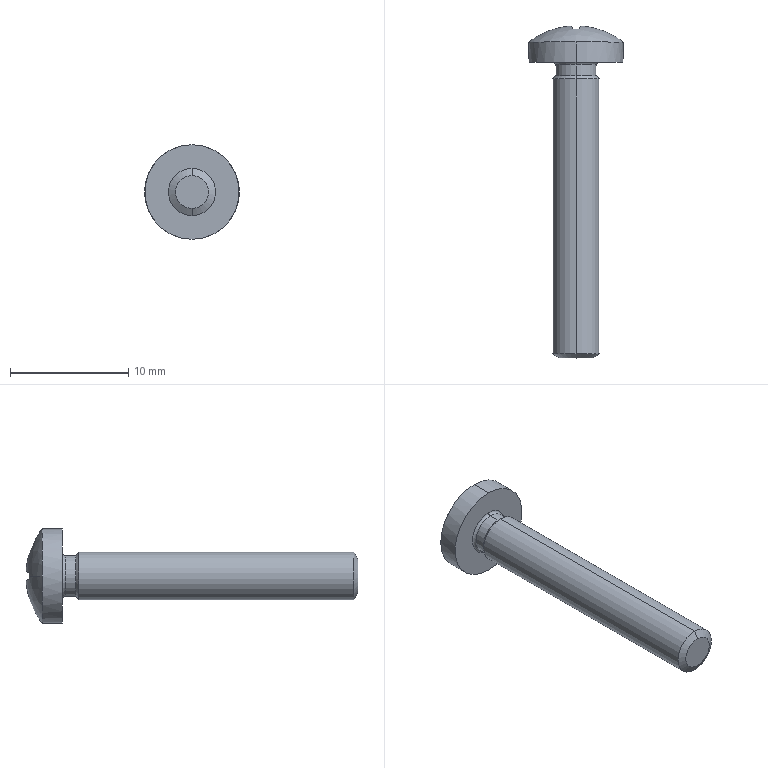Component | SolidWorks | GB_T818-2000PhillipsPanHeadScrewM4_25-1 | 1 solid | 28 faces | box 8 x 28.08 x 8 mm | volume 428 mm3 | plane 14 | cylinder 6 | cone 4 | torus 2 | sphere 2 | commonest cylinder face diameters 3.464 x2 8 x2 4 x2
build123d program:
from build123d import *


with BuildPart() as part:
    # Sketch2 → Base-Revolve (revolve)
    with BuildSketch(Plane.XY, mode=Mode.PRIVATE) as base_revolve_sk:
        with BuildLine():
            Line((0, 0), (28.1, 0))
            Line((28.1, 0), (28.1, 2))
            Line((28.1, 2), (4.5, 2))
            Line((4.5, 2), (4.232, 1.732))
            Line((4.232, 1.732), (3.318, 1.732))
            ThreePointArc((3.318, 1.732), (3.164, 1.796), (3.1, 1.95))
            Line((3.1, 1.95), (3.1, 4))
            Line((3.1, 4), (1.377, 4))
            ThreePointArc((1.377, 4), (0.3538, 2.115), (0, 0))
        make_face()
    revolve(base_revolve_sk.sketch.rotate(Axis((-1.332, 0, 0), (1, 0, 0)), 90), axis=Axis((-1.332, 0, 0), (1, 0, 0)))

    # Sketch3 → Cut-Revolve1 (revolve, cut)
    with BuildSketch(Plane.XY, mode=Mode.PRIVATE) as cut_revolve1_sk:
        Polygon((27.754, 2), (28.454, 2), (28.1, 1.394), align=None)
    revolve(cut_revolve1_sk.sketch.rotate(Axis((-0.2428, 0, 0), (1, 0, 0)), 90), axis=Axis((-0.2428, 0, 0), (1, 0, 0)), mode=Mode.SUBTRACT)

    # Sketch5 → Cut-Loft1 section 0
    with BuildSketch(Plane(origin=(0, 0, 0), x_dir=(0, 0, -1), z_dir=(1, 0, 0)), mode=Mode.PRIVATE) as cut_loft1_s0:
        with BuildLine():
            Line((0.35, 2.2), (-0.35, 2.2))
            Line((-0.35, 2.2), (-0.35, -2.2))
            Line((-0.35, -2.2), (0.35, -2.2))
            Line((0.35, -2.2), (0.35, 2.2))
        make_face()
    cut_loft1 = loft([Vertex(2.4, 0, 0), cut_loft1_s0.sketch], mode=Mode.SUBTRACT)

    # Mirror1: Cut-Loft1 across plane
    add(cut_loft1.mirror(Plane(origin=(0, 0, 0), x_dir=(0, 0.7071, 0.7071), z_dir=(0, -0.7071, 0.7071))), mode=Mode.SUBTRACT)


solid = part.part

# Placed as in the assembly
solid = solid.moved(Location((-130.534, 135.266, -166.507), (0, 0, -90)))
STEP:
#1=COLOUR_RGB('',0.7922,0.8196,0.9333);
#2=FILL_AREA_STYLE_COLOUR('',#1);
#3=FILL_AREA_STYLE('',(#2));
#4=SURFACE_STYLE_FILL_AREA(#3);
#5=SURFACE_SIDE_STYLE('',(#4));
#6=SURFACE_STYLE_USAGE(.BOTH.,#5);
#7=PRESENTATION_STYLE_ASSIGNMENT((#6));
#8=CARTESIAN_POINT('',(-5.139,4.219,-6.501));
#9=VERTEX_POINT('',#8);
#10=CARTESIAN_POINT('',(-5.139,4.219,-6.61));
#11=VERTEX_POINT('',#10);
#12=CARTESIAN_POINT('',(-5.139,4.219,-6.555));
#13=DIRECTION('',(0.,1.,0.));
#14=DIRECTION('',(0.,0.,1.));
#15=AXIS2_PLACEMENT_3D('',#12,#13,#14);
#16=CIRCLE('',#15,0.05487);
#17=EDGE_CURVE('',#9,#11,#16,.T.);
#18=ORIENTED_EDGE('',*,*,#17,.T.);
#19=CARTESIAN_POINT('',(-5.139,4.233,-6.634));
#20=VERTEX_POINT('',#19);
#21=CARTESIAN_POINT('',(-5.139,4.233,-6.634));
#22=DIRECTION('',(0.,0.4959,-0.8684));
#23=VECTOR('',#22,39.37);
#24=LINE('',#21,#23);
#25=EDGE_CURVE('',#11,#20,#24,.T.);
#26=ORIENTED_EDGE('',*,*,#25,.T.);
#27=CARTESIAN_POINT('',(-5.139,4.233,-6.477));
#28=VERTEX_POINT('',#27);
#29=CARTESIAN_POINT('',(-5.139,4.233,-6.555));
#30=DIRECTION('',(0.,1.,0.));
#31=DIRECTION('',(0.,0.,1.));
#32=AXIS2_PLACEMENT_3D('',#29,#30,#31);
#33=CIRCLE('',#32,0.07874);
#34=EDGE_CURVE('',#28,#20,#33,.T.);
#35=ORIENTED_EDGE('',*,*,#34,.F.);
#36=CARTESIAN_POINT('',(-5.139,4.233,-6.477));
#37=DIRECTION('',(0.,0.4959,0.8684));
#38=VECTOR('',#37,39.37);
#39=LINE('',#36,#38);
#40=EDGE_CURVE('',#9,#28,#39,.T.);
#41=ORIENTED_EDGE('',*,*,#40,.F.);
#42=EDGE_LOOP('',(#18,#26,#35,#41));
#43=FACE_OUTER_BOUND('',#42,.T.);
#44=CARTESIAN_POINT('',(-5.139,4.233,-6.555));
#45=DIRECTION('',(0.,1.,0.));
#46=DIRECTION('',(0.,0.,1.));
#47=AXIS2_PLACEMENT_3D('',#44,#45,#46);
#48=CONICAL_SURFACE('',#47,0.07874,1.052);
#49=ADVANCED_FACE('',(#43),#48,.T.);
#50=CARTESIAN_POINT('',(-5.139,5.159,-6.487));
#51=VERTEX_POINT('',#50);
#52=CARTESIAN_POINT('',(-5.139,5.159,-6.624));
#53=VERTEX_POINT('',#52);
#54=CARTESIAN_POINT('',(-5.139,5.159,-6.555));
#55=DIRECTION('',(0.,1.,0.));
#56=DIRECTION('',(0.,0.,1.));
#57=AXIS2_PLACEMENT_3D('',#54,#55,#56);
#58=CIRCLE('',#57,0.06819);
#59=EDGE_CURVE('',#51,#53,#58,.T.);
#60=ORIENTED_EDGE('',*,*,#59,.F.);
#61=CARTESIAN_POINT('',(-5.139,5.148,-6.477));
#62=VERTEX_POINT('',#61);
#63=CARTESIAN_POINT('',(-5.139,5.148,-6.477));
#64=DIRECTION('',(0.,-0.7071,0.7071));
#65=VECTOR('',#64,39.37);
#66=LINE('',#63,#65);
#67=EDGE_CURVE('',#51,#62,#66,.T.);
#68=ORIENTED_EDGE('',*,*,#67,.T.);
#69=CARTESIAN_POINT('',(-5.139,5.148,-6.634));
#70=VERTEX_POINT('',#69);
#71=CARTESIAN_POINT('',(-5.139,5.148,-6.555));
#72=DIRECTION('',(0.,1.,0.));
#73=DIRECTION('',(0.,0.,1.));
#74=AXIS2_PLACEMENT_3D('',#71,#72,#73);
#75=CIRCLE('',#74,0.07874);
#76=EDGE_CURVE('',#62,#70,#75,.T.);
#77=ORIENTED_EDGE('',*,*,#76,.T.);
#78=CARTESIAN_POINT('',(-5.139,5.148,-6.634));
#79=DIRECTION('',(0.,-0.7071,-0.7071));
#80=VECTOR('',#79,39.37);
#81=LINE('',#78,#80);
#82=EDGE_CURVE('',#53,#70,#81,.T.);
#83=ORIENTED_EDGE('',*,*,#82,.F.);
#84=EDGE_LOOP('',(#60,#68,#77,#83));
#85=FACE_OUTER_BOUND('',#84,.T.);
#86=CARTESIAN_POINT('',(-5.139,5.148,-6.555));
#87=DIRECTION('',(0.,-1.,0.));
#88=DIRECTION('',(0.,0.,-1.));
#89=AXIS2_PLACEMENT_3D('',#86,#87,#88);
#90=CONICAL_SURFACE('',#89,0.07874,0.7854);
#91=ADVANCED_FACE('',(#85),#90,.T.);
#92=ORIENTED_EDGE('',*,*,#59,.T.);
#93=CARTESIAN_POINT('',(-5.139,5.195,-6.624));
#94=VERTEX_POINT('',#93);
#95=CARTESIAN_POINT('',(-5.139,5.378,-6.624));
#96=DIRECTION('',(0.,1.,0.));
#97=VECTOR('',#96,39.37);
#98=LINE('',#95,#97);
#99=EDGE_CURVE('',#53,#94,#98,.T.);
#100=ORIENTED_EDGE('',*,*,#99,.T.);
#101=CARTESIAN_POINT('',(-5.139,5.195,-6.487));
#102=VERTEX_POINT('',#101);
#103=CARTESIAN_POINT('',(-5.139,5.195,-6.555));
#104=DIRECTION('',(0.,1.,0.));
#105=DIRECTION('',(0.,0.,1.));
#106=AXIS2_PLACEMENT_3D('',#103,#104,#105);
#107=CIRCLE('',#106,0.06819);
#108=EDGE_CURVE('',#102,#94,#107,.T.);
#109=ORIENTED_EDGE('',*,*,#108,.F.);
#110=CARTESIAN_POINT('',(-5.139,5.378,-6.487));
#111=DIRECTION('',(0.,1.,0.));
#112=VECTOR('',#111,39.37);
#113=LINE('',#110,#112);
#114=EDGE_CURVE('',#51,#102,#113,.T.);
#115=ORIENTED_EDGE('',*,*,#114,.F.);
#116=EDGE_LOOP('',(#92,#100,#109,#115));
#117=FACE_OUTER_BOUND('',#116,.T.);
#118=CARTESIAN_POINT('',(-5.139,5.378,-6.555));
#119=DIRECTION('',(0.,1.,0.));
#120=DIRECTION('',(0.,0.,1.));
#121=AXIS2_PLACEMENT_3D('',#118,#119,#120);
#122=CYLINDRICAL_SURFACE('',#121,0.06819);
#123=ADVANCED_FACE('',(#117),#122,.T.);
#124=CARTESIAN_POINT('',(-5.139,5.203,-6.632));
#125=VERTEX_POINT('',#124);
#126=CARTESIAN_POINT('',(-5.139,5.203,-6.479));
#127=VERTEX_POINT('',#126);
#128=CARTESIAN_POINT('',(-5.139,5.203,-6.555));
#129=DIRECTION('',(0.,1.,0.));
#130=DIRECTION('',(0.,0.,1.));
#131=AXIS2_PLACEMENT_3D('',#128,#129,#130);
#132=CIRCLE('',#131,0.07677);
#133=EDGE_CURVE('',#125,#127,#132,.T.);
#134=ORIENTED_EDGE('',*,*,#133,.F.);
#135=CARTESIAN_POINT('',(-5.139,5.195,-6.632));
#136=DIRECTION('',(1.,0.,0.));
#137=DIRECTION('',(0.,0.,-1.));
#138=AXIS2_PLACEMENT_3D('',#135,#136,#137);
#139=CIRCLE('',#138,0.008583);
#140=EDGE_CURVE('',#125,#94,#139,.T.);
#141=ORIENTED_EDGE('',*,*,#140,.T.);
#142=CARTESIAN_POINT('',(-5.139,5.195,-6.555));
#143=DIRECTION('',(0.,1.,0.));
#144=DIRECTION('',(0.,0.,1.));
#145=AXIS2_PLACEMENT_3D('',#142,#143,#144);
#146=CIRCLE('',#145,0.06819);
#147=EDGE_CURVE('',#94,#102,#146,.T.);
#148=ORIENTED_EDGE('',*,*,#147,.T.);
#149=CARTESIAN_POINT('',(-5.139,5.195,-6.479));
#150=DIRECTION('',(-1.,0.,0.));
#151=DIRECTION('',(0.,0.,1.));
#152=AXIS2_PLACEMENT_3D('',#149,#150,#151);
#153=CIRCLE('',#152,0.008583);
#154=EDGE_CURVE('',#127,#102,#153,.T.);
#155=ORIENTED_EDGE('',*,*,#154,.F.);
#156=EDGE_LOOP('',(#134,#141,#148,#155));
#157=FACE_OUTER_BOUND('',#156,.T.);
#158=CARTESIAN_POINT('',(-5.139,5.195,-6.555));
#159=DIRECTION('',(0.,1.,0.));
#160=DIRECTION('',(0.,0.,1.));
#161=AXIS2_PLACEMENT_3D('',#158,#159,#160);
#162=TOROIDAL_SURFACE('',#161,0.07677,0.008583);
#163=ADVANCED_FACE('',(#157),#162,.F.);
#164=CARTESIAN_POINT('',(-5.139,5.203,-6.398));
#165=VERTEX_POINT('',#164);
#166=CARTESIAN_POINT('',(-5.139,5.203,-6.713));
#167=VERTEX_POINT('',#166);
#168=CARTESIAN_POINT('',(-5.139,5.203,-6.555));
#169=DIRECTION('',(0.,1.,0.));
#170=DIRECTION('',(0.,0.,1.));
#171=AXIS2_PLACEMENT_3D('',#168,#169,#170);
#172=CIRCLE('',#171,0.1575);
#173=EDGE_CURVE('',#165,#167,#172,.T.);
#174=ORIENTED_EDGE('',*,*,#173,.T.);
#175=CARTESIAN_POINT('',(-5.139,5.271,-6.713));
#176=VERTEX_POINT('',#175);
#177=CARTESIAN_POINT('',(-5.139,5.378,-6.713));
#178=DIRECTION('',(0.,1.,0.));
#179=VECTOR('',#178,39.37);
#180=LINE('',#177,#179);
#181=EDGE_CURVE('',#167,#176,#180,.T.);
#182=ORIENTED_EDGE('',*,*,#181,.T.);
#183=CARTESIAN_POINT('',(-4.982,5.271,-6.555));
#184=VERTEX_POINT('',#183);
#185=CARTESIAN_POINT('',(-5.139,5.271,-6.555));
#186=DIRECTION('',(0.,1.,0.));
#187=DIRECTION('',(0.,0.,1.));
#188=AXIS2_PLACEMENT_3D('',#185,#186,#187);
#189=CIRCLE('',#188,0.1575);
#190=EDGE_CURVE('',#184,#176,#189,.T.);
#191=ORIENTED_EDGE('',*,*,#190,.F.);
#192=CARTESIAN_POINT('',(-5.139,5.271,-6.398));
#193=VERTEX_POINT('',#192);
#194=CARTESIAN_POINT('',(-5.139,5.271,-6.555));
#195=DIRECTION('',(0.,1.,0.));
#196=DIRECTION('',(0.,0.,1.));
#197=AXIS2_PLACEMENT_3D('',#194,#195,#196);
#198=CIRCLE('',#197,0.1575);
#199=EDGE_CURVE('',#193,#184,#198,.T.);
#200=ORIENTED_EDGE('',*,*,#199,.F.);
#201=CARTESIAN_POINT('',(-5.139,5.378,-6.398));
#202=DIRECTION('',(0.,1.,0.));
#203=VECTOR('',#202,39.37);
#204=LINE('',#201,#203);
#205=EDGE_CURVE('',#165,#193,#204,.T.);
#206=ORIENTED_EDGE('',*,*,#205,.F.);
#207=EDGE_LOOP('',(#174,#182,#191,#200,#206));
#208=FACE_OUTER_BOUND('',#207,.T.);
#209=CARTESIAN_POINT('',(-5.139,5.378,-6.555));
#210=DIRECTION('',(0.,1.,0.));
#211=DIRECTION('',(0.,0.,1.));
#212=AXIS2_PLACEMENT_3D('',#209,#210,#211);
#213=CYLINDRICAL_SURFACE('',#212,0.1575);
#214=ADVANCED_FACE('',(#208),#213,.T.);
#215=ORIENTED_EDGE('',*,*,#190,.T.);
#216=CARTESIAN_POINT('',(-5.297,5.271,-6.555));
#217=VERTEX_POINT('',#216);
#218=CARTESIAN_POINT('',(-5.139,5.271,-6.555));
#219=DIRECTION('',(0.,1.,0.));
#220=DIRECTION('',(0.,0.,1.));
#221=AXIS2_PLACEMENT_3D('',#218,#219,#220);
#222=CIRCLE('',#221,0.1575);
#223=EDGE_CURVE('',#176,#217,#222,.T.);
#224=ORIENTED_EDGE('',*,*,#223,.T.);
#225=CARTESIAN_POINT('',(-5.215,5.314,-6.555));
#226=VERTEX_POINT('',#225);
#227=CARTESIAN_POINT('',(-5.139,5.07,-6.555));
#228=DIRECTION('',(0.,0.,-1.));
#229=DIRECTION('',(-1.,0.,0.));
#230=AXIS2_PLACEMENT_3D('',#227,#228,#229);
#231=CIRCLE('',#230,0.2559);
#232=EDGE_CURVE('',#217,#226,#231,.T.);
#233=ORIENTED_EDGE('',*,*,#232,.T.);
#234=CARTESIAN_POINT('',(-5.215,5.314,-6.567));
#235=VERTEX_POINT('',#234);
#236=CARTESIAN_POINT('',(-5.059,5.143,-6.555));
#237=DIRECTION('',(-0.7372,-0.6757,0.));
#238=DIRECTION('',(0.6757,-0.7372,0.));
#239=AXIS2_PLACEMENT_3D('',#236,#237,#238);
#240=CIRCLE('',#239,0.2315);
#241=EDGE_CURVE('',#226,#235,#240,.T.);
#242=ORIENTED_EDGE('',*,*,#241,.T.);
#243=CARTESIAN_POINT('',(-5.153,5.325,-6.569));
#244=VERTEX_POINT('',#243);
#245=CARTESIAN_POINT('',(-5.139,5.073,-6.532));
#246=DIRECTION('',(0.,-0.1443,-0.9895));
#247=DIRECTION('',(0.,0.9895,-0.1443));
#248=AXIS2_PLACEMENT_3D('',#245,#246,#247);
#249=CIRCLE('',#248,0.2548);
#250=EDGE_CURVE('',#235,#244,#249,.T.);
#251=ORIENTED_EDGE('',*,*,#250,.T.);
#252=CARTESIAN_POINT('',(-5.151,5.314,-6.631));
#253=VERTEX_POINT('',#252);
#254=CARTESIAN_POINT('',(-5.116,5.073,-6.555));
#255=DIRECTION('',(-0.9895,-0.1443,-0.));
#256=DIRECTION('',(0.1443,-0.9895,0.));
#257=AXIS2_PLACEMENT_3D('',#254,#255,#256);
#258=CIRCLE('',#257,0.2548);
#259=EDGE_CURVE('',#244,#253,#258,.T.);
#260=ORIENTED_EDGE('',*,*,#259,.T.);
#261=CARTESIAN_POINT('',(-5.127,5.314,-6.631));
#262=VERTEX_POINT('',#261);
#263=CARTESIAN_POINT('',(-5.139,5.143,-6.475));
#264=DIRECTION('',(0.,-0.6757,-0.7372));
#265=DIRECTION('',(0.,0.7372,-0.6757));
#266=AXIS2_PLACEMENT_3D('',#263,#264,#265);
#267=CIRCLE('',#266,0.2315);
#268=EDGE_CURVE('',#253,#262,#267,.T.);
#269=ORIENTED_EDGE('',*,*,#268,.T.);
#270=CARTESIAN_POINT('',(-5.125,5.325,-6.569));
#271=VERTEX_POINT('',#270);
#272=CARTESIAN_POINT('',(-5.162,5.073,-6.555));
#273=DIRECTION('',(0.9895,-0.1443,0.));
#274=DIRECTION('',(0.1443,0.9895,0.));
#275=AXIS2_PLACEMENT_3D('',#272,#273,#274);
#276=CIRCLE('',#275,0.2548);
#277=EDGE_CURVE('',#262,#271,#276,.T.);
#278=ORIENTED_EDGE('',*,*,#277,.T.);
#279=CARTESIAN_POINT('',(-5.063,5.314,-6.567));
#280=VERTEX_POINT('',#279);
#281=CARTESIAN_POINT('',(-5.139,5.073,-6.532));
#282=DIRECTION('',(0.,-0.1443,-0.9895));
#283=DIRECTION('',(0.,0.9895,-0.1443));
#284=AXIS2_PLACEMENT_3D('',#281,#282,#283);
#285=CIRCLE('',#284,0.2548);
#286=EDGE_CURVE('',#271,#280,#285,.T.);
#287=ORIENTED_EDGE('',*,*,#286,.T.);
#288=CARTESIAN_POINT('',(-5.063,5.314,-6.555));
#289=VERTEX_POINT('',#288);
#290=CARTESIAN_POINT('',(-5.22,5.143,-6.555));
#291=DIRECTION('',(0.7372,-0.6757,0.));
#292=DIRECTION('',(0.6757,0.7372,0.));
#293=AXIS2_PLACEMENT_3D('',#290,#291,#292);
#294=CIRCLE('',#293,0.2315);
#295=EDGE_CURVE('',#280,#289,#294,.T.);
#296=ORIENTED_EDGE('',*,*,#295,.T.);
#297=CARTESIAN_POINT('',(-5.139,5.07,-6.555));
#298=DIRECTION('',(0.,0.,1.));
#299=DIRECTION('',(1.,0.,0.));
#300=AXIS2_PLACEMENT_3D('',#297,#298,#299);
#301=CIRCLE('',#300,0.2559);
#302=EDGE_CURVE('',#184,#289,#301,.T.);
#303=ORIENTED_EDGE('',*,*,#302,.F.);
#304=EDGE_LOOP('',(#215,#224,#233,#242,#251,#260,#269,#278,#287,#296,#303));
#305=FACE_OUTER_BOUND('',#304,.T.);
#306=CARTESIAN_POINT('',(-5.139,5.07,-6.555));
#307=DIRECTION('',(0.,0.,-1.));
#308=DIRECTION('',(1.,0.,0.));
#309=AXIS2_PLACEMENT_3D('',#306,#307,#308);
#310=SPHERICAL_SURFACE('',#309,0.2559);
#311=ADVANCED_FACE('',(#305),#310,.T.);
#312=ORIENTED_EDGE('',*,*,#34,.T.);
#313=CARTESIAN_POINT('',(-5.139,5.378,-6.634));
#314=DIRECTION('',(0.,1.,0.));
#315=VECTOR('',#314,39.37);
#316=LINE('',#313,#315);
#317=EDGE_CURVE('',#20,#70,#316,.T.);
#318=ORIENTED_EDGE('',*,*,#317,.T.);
#319=ORIENTED_EDGE('',*,*,#76,.F.);
#320=CARTESIAN_POINT('',(-5.139,5.378,-6.477));
#321=DIRECTION('',(0.,1.,0.));
#322=VECTOR('',#321,39.37);
#323=LINE('',#320,#322);
#324=EDGE_CURVE('',#28,#62,#323,.T.);
#325=ORIENTED_EDGE('',*,*,#324,.F.);
#326=EDGE_LOOP('',(#312,#318,#319,#325));
#327=FACE_OUTER_BOUND('',#326,.T.);
#328=CARTESIAN_POINT('',(-5.139,5.378,-6.555));
#329=DIRECTION('',(0.,1.,0.));
#330=DIRECTION('',(0.,0.,1.));
#331=AXIS2_PLACEMENT_3D('',#328,#329,#330);
#332=CYLINDRICAL_SURFACE('',#331,0.07874);
#333=ADVANCED_FACE('',(#327),#332,.T.);
#334=CARTESIAN_POINT('',(-5.139,5.231,-6.555));
#335=VERTEX_POINT('',#334);
#336=CARTESIAN_POINT('',(-5.139,5.231,-6.555));
#337=DIRECTION('',(-0.6719,0.7329,-0.1069));
#338=VECTOR('',#337,39.37);
#339=LINE('',#336,#338);
#340=EDGE_CURVE('',#335,#235,#339,.T.);
#341=ORIENTED_EDGE('',*,*,#340,.F.);
#342=CARTESIAN_POINT('',(-5.139,5.231,-6.555));
#343=DIRECTION('',(-0.1428,0.9794,-0.1428));
#344=VECTOR('',#343,39.37);
#345=LINE('',#342,#344);
#346=EDGE_CURVE('',#335,#244,#345,.T.);
#347=ORIENTED_EDGE('',*,*,#346,.T.);
#348=ORIENTED_EDGE('',*,*,#250,.F.);
#349=EDGE_LOOP('',(#341,#347,#348));
#350=FACE_OUTER_BOUND('',#349,.T.);
#351=CARTESIAN_POINT('',(-5.139,5.231,-6.555));
#352=DIRECTION('',(0.,-0.1443,-0.9895));
#353=DIRECTION('',(0.,0.9895,-0.1443));
#354=AXIS2_PLACEMENT_3D('',#351,#352,#353);
#355=PLANE('',#354);
#356=ADVANCED_FACE('',(#350),#355,.F.);
#357=CARTESIAN_POINT('',(-5.153,5.325,-6.542));
#358=VERTEX_POINT('',#357);
#359=CARTESIAN_POINT('',(-5.215,5.314,-6.543));
#360=VERTEX_POINT('',#359);
#361=CARTESIAN_POINT('',(-5.139,5.073,-6.578));
#362=DIRECTION('',(0.,-0.1443,0.9895));
#363=DIRECTION('',(0.,-0.9895,-0.1443));
#364=AXIS2_PLACEMENT_3D('',#361,#362,#363);
#365=CIRCLE('',#364,0.2548);
#366=EDGE_CURVE('',#358,#360,#365,.T.);
#367=ORIENTED_EDGE('',*,*,#366,.F.);
#368=CARTESIAN_POINT('',(-5.139,5.231,-6.555));
#369=DIRECTION('',(0.1428,-0.9794,-0.1428));
#370=VECTOR('',#369,39.37);
#371=LINE('',#368,#370);
#372=EDGE_CURVE('',#358,#335,#371,.T.);
#373=ORIENTED_EDGE('',*,*,#372,.T.);
#374=CARTESIAN_POINT('',(-5.139,5.231,-6.555));
#375=DIRECTION('',(-0.6719,0.7329,0.1069));
#376=VECTOR('',#375,39.37);
#377=LINE('',#374,#376);
#378=EDGE_CURVE('',#335,#360,#377,.T.);
#379=ORIENTED_EDGE('',*,*,#378,.T.);
#380=EDGE_LOOP('',(#367,#373,#379));
#381=FACE_OUTER_BOUND('',#380,.T.);
#382=CARTESIAN_POINT('',(-5.139,5.231,-6.555));
#383=DIRECTION('',(0.,-0.1443,0.9895));
#384=DIRECTION('',(0.,-0.9895,-0.1443));
#385=AXIS2_PLACEMENT_3D('',#382,#383,#384);
#386=PLANE('',#385);
#387=ADVANCED_FACE('',(#381),#386,.F.);
#388=ORIENTED_EDGE('',*,*,#317,.F.);
#389=CARTESIAN_POINT('',(-5.139,4.233,-6.555));
#390=DIRECTION('',(0.,1.,0.));
#391=DIRECTION('',(0.,0.,1.));
#392=AXIS2_PLACEMENT_3D('',#389,#390,#391);
#393=CIRCLE('',#392,0.07874);
#394=EDGE_CURVE('',#20,#28,#393,.T.);
#395=ORIENTED_EDGE('',*,*,#394,.T.);
#396=ORIENTED_EDGE('',*,*,#324,.T.);
#397=CARTESIAN_POINT('',(-5.139,5.148,-6.555));
#398=DIRECTION('',(0.,1.,0.));
#399=DIRECTION('',(0.,0.,1.));
#400=AXIS2_PLACEMENT_3D('',#397,#398,#399);
#401=CIRCLE('',#400,0.07874);
#402=EDGE_CURVE('',#70,#62,#401,.T.);
#403=ORIENTED_EDGE('',*,*,#402,.F.);
#404=EDGE_LOOP('',(#388,#395,#396,#403));
#405=FACE_OUTER_BOUND('',#404,.T.);
#406=CARTESIAN_POINT('',(-5.139,5.378,-6.555));
#407=DIRECTION('',(0.,1.,0.));
#408=DIRECTION('',(0.,0.,1.));
#409=AXIS2_PLACEMENT_3D('',#406,#407,#408);
#410=CYLINDRICAL_SURFACE('',#409,0.07874);
#411=ADVANCED_FACE('',(#405),#410,.T.);
#412=ORIENTED_EDGE('',*,*,#232,.F.);
#413=CARTESIAN_POINT('',(-5.139,5.271,-6.555));
#414=DIRECTION('',(0.,1.,0.));
#415=DIRECTION('',(0.,0.,1.));
#416=AXIS2_PLACEMENT_3D('',#413,#414,#415);
#417=CIRCLE('',#416,0.1575);
#418=EDGE_CURVE('',#217,#193,#417,.T.);
#419=ORIENTED_EDGE('',*,*,#418,.T.);
#420=ORIENTED_EDGE('',*,*,#199,.T.);
#421=ORIENTED_EDGE('',*,*,#302,.T.);
#422=CARTESIAN_POINT('',(-5.063,5.314,-6.543));
#423=VERTEX_POINT('',#422);
#424=CARTESIAN_POINT('',(-5.22,5.143,-6.555));
#425=DIRECTION('',(0.7372,-0.6757,0.));
#426=DIRECTION('',(0.6757,0.7372,0.));
#427=AXIS2_PLACEMENT_3D('',#424,#425,#426);
#428=CIRCLE('',#427,0.2315);
#429=EDGE_CURVE('',#289,#423,#428,.T.);
#430=ORIENTED_EDGE('',*,*,#429,.T.);
#431=CARTESIAN_POINT('',(-5.125,5.325,-6.542));
#432=VERTEX_POINT('',#431);
#433=CARTESIAN_POINT('',(-5.139,5.073,-6.578));
#434=DIRECTION('',(0.,-0.1443,0.9895));
#435=DIRECTION('',(0.,-0.9895,-0.1443));
#436=AXIS2_PLACEMENT_3D('',#433,#434,#435);
#437=CIRCLE('',#436,0.2548);
#438=EDGE_CURVE('',#423,#432,#437,.T.);
#439=ORIENTED_EDGE('',*,*,#438,.T.);
#440=CARTESIAN_POINT('',(-5.127,5.314,-6.48));
#441=VERTEX_POINT('',#440);
#442=CARTESIAN_POINT('',(-5.162,5.073,-6.555));
#443=DIRECTION('',(0.9895,-0.1443,0.));
#444=DIRECTION('',(0.1443,0.9895,0.));
#445=AXIS2_PLACEMENT_3D('',#442,#443,#444);
#446=CIRCLE('',#445,0.2548);
#447=EDGE_CURVE('',#432,#441,#446,.T.);
#448=ORIENTED_EDGE('',*,*,#447,.T.);
#449=CARTESIAN_POINT('',(-5.151,5.314,-6.48));
#450=VERTEX_POINT('',#449);
#451=CARTESIAN_POINT('',(-5.139,5.143,-6.636));
#452=DIRECTION('',(-0.,-0.6757,0.7372));
#453=DIRECTION('',(0.,-0.7372,-0.6757));
#454=AXIS2_PLACEMENT_3D('',#451,#452,#453);
#455=CIRCLE('',#454,0.2315);
#456=EDGE_CURVE('',#441,#450,#455,.T.);
#457=ORIENTED_EDGE('',*,*,#456,.T.);
#458=CARTESIAN_POINT('',(-5.116,5.073,-6.555));
#459=DIRECTION('',(-0.9895,-0.1443,-0.));
#460=DIRECTION('',(0.1443,-0.9895,0.));
#461=AXIS2_PLACEMENT_3D('',#458,#459,#460);
#462=CIRCLE('',#461,0.2548);
#463=EDGE_CURVE('',#450,#358,#462,.T.);
#464=ORIENTED_EDGE('',*,*,#463,.T.);
#465=ORIENTED_EDGE('',*,*,#366,.T.);
#466=CARTESIAN_POINT('',(-5.059,5.143,-6.555));
#467=DIRECTION('',(-0.7372,-0.6757,0.));
#468=DIRECTION('',(0.6757,-0.7372,0.));
#469=AXIS2_PLACEMENT_3D('',#466,#467,#468);
#470=CIRCLE('',#469,0.2315);
#471=EDGE_CURVE('',#360,#226,#470,.T.);
#472=ORIENTED_EDGE('',*,*,#471,.T.);
#473=EDGE_LOOP('',(#412,#419,#420,#421,#430,#439,#448,#457,#464,#465,#472));
#474=FACE_OUTER_BOUND('',#473,.T.);
#475=CARTESIAN_POINT('',(-5.139,5.07,-6.555));
#476=DIRECTION('',(0.,0.,-1.));
#477=DIRECTION('',(1.,0.,0.));
#478=AXIS2_PLACEMENT_3D('',#475,#476,#477);
#479=SPHERICAL_SURFACE('',#478,0.2559);
#480=ADVANCED_FACE('',(#474),#479,.T.);
#481=ORIENTED_EDGE('',*,*,#181,.F.);
#482=CARTESIAN_POINT('',(-5.139,5.203,-6.555));
#483=DIRECTION('',(0.,1.,0.));
#484=DIRECTION('',(0.,0.,1.));
#485=AXIS2_PLACEMENT_3D('',#482,#483,#484);
#486=CIRCLE('',#485,0.1575);
#487=EDGE_CURVE('',#167,#165,#486,.T.);
#488=ORIENTED_EDGE('',*,*,#487,.T.);
#489=ORIENTED_EDGE('',*,*,#205,.T.);
#490=ORIENTED_EDGE('',*,*,#418,.F.);
#491=ORIENTED_EDGE('',*,*,#223,.F.);
#492=EDGE_LOOP('',(#481,#488,#489,#490,#491));
#493=FACE_OUTER_BOUND('',#492,.T.);
#494=CARTESIAN_POINT('',(-5.139,5.378,-6.555));
#495=DIRECTION('',(0.,1.,0.));
#496=DIRECTION('',(0.,0.,1.));
#497=AXIS2_PLACEMENT_3D('',#494,#495,#496);
#498=CYLINDRICAL_SURFACE('',#497,0.1575);
#499=ADVANCED_FACE('',(#493),#498,.T.);
#500=ORIENTED_EDGE('',*,*,#173,.F.);
#501=ORIENTED_EDGE('',*,*,#487,.F.);
#502=EDGE_LOOP('',(#500,#501));
#503=FACE_OUTER_BOUND('',#502,.T.);
#504=CARTESIAN_POINT('',(-5.139,5.203,-6.555));
#505=DIRECTION('',(0.,1.,0.));
#506=DIRECTION('',(0.,0.,1.));
#507=AXIS2_PLACEMENT_3D('',#504,#505,#506);
#508=CIRCLE('',#507,0.07677);
#509=EDGE_CURVE('',#127,#125,#508,.T.);
#510=ORIENTED_EDGE('',*,*,#509,.T.);
#511=ORIENTED_EDGE('',*,*,#133,.T.);
#512=EDGE_LOOP('',(#510,#511));
#513=FACE_BOUND('',#512,.T.);
#514=CARTESIAN_POINT('',(-5.062,5.203,-6.555));
#515=DIRECTION('',(0.,1.,0.));
#516=DIRECTION('',(0.,0.,1.));
#517=AXIS2_PLACEMENT_3D('',#514,#515,#516);
#518=PLANE('',#517);
#519=ADVANCED_FACE('',(#503,#513),#518,.F.);
#520=ORIENTED_EDGE('',*,*,#140,.F.);
#521=ORIENTED_EDGE('',*,*,#509,.F.);
#522=ORIENTED_EDGE('',*,*,#154,.T.);
#523=ORIENTED_EDGE('',*,*,#108,.T.);
#524=EDGE_LOOP('',(#520,#521,#522,#523));
#525=FACE_OUTER_BOUND('',#524,.T.);
#526=CARTESIAN_POINT('',(-5.139,5.195,-6.555));
#527=DIRECTION('',(0.,1.,0.));
#528=DIRECTION('',(0.,0.,1.));
#529=AXIS2_PLACEMENT_3D('',#526,#527,#528);
#530=TOROIDAL_SURFACE('',#529,0.07677,0.008583);
#531=ADVANCED_FACE('',(#525),#530,.F.);
#532=ORIENTED_EDGE('',*,*,#99,.F.);
#533=CARTESIAN_POINT('',(-5.139,5.159,-6.555));
#534=DIRECTION('',(0.,1.,0.));
#535=DIRECTION('',(0.,0.,1.));
#536=AXIS2_PLACEMENT_3D('',#533,#534,#535);
#537=CIRCLE('',#536,0.06819);
#538=EDGE_CURVE('',#53,#51,#537,.T.);
#539=ORIENTED_EDGE('',*,*,#538,.T.);
#540=ORIENTED_EDGE('',*,*,#114,.T.);
#541=ORIENTED_EDGE('',*,*,#147,.F.);
#542=EDGE_LOOP('',(#532,#539,#540,#541));
#543=FACE_OUTER_BOUND('',#542,.T.);
#544=CARTESIAN_POINT('',(-5.139,5.378,-6.555));
#545=DIRECTION('',(0.,1.,0.));
#546=DIRECTION('',(0.,0.,1.));
#547=AXIS2_PLACEMENT_3D('',#544,#545,#546);
#548=CYLINDRICAL_SURFACE('',#547,0.06819);
#549=ADVANCED_FACE('',(#543),#548,.T.);
#550=ORIENTED_EDGE('',*,*,#67,.F.);
#551=ORIENTED_EDGE('',*,*,#538,.F.);
#552=ORIENTED_EDGE('',*,*,#82,.T.);
#553=ORIENTED_EDGE('',*,*,#402,.T.);
#554=EDGE_LOOP('',(#550,#551,#552,#553));
#555=FACE_OUTER_BOUND('',#554,.T.);
#556=CARTESIAN_POINT('',(-5.139,5.148,-6.555));
#557=DIRECTION('',(0.,-1.,0.));
#558=DIRECTION('',(0.,0.,-1.));
#559=AXIS2_PLACEMENT_3D('',#556,#557,#558);
#560=CONICAL_SURFACE('',#559,0.07874,0.7854);
#561=ADVANCED_FACE('',(#555),#560,.T.);
#562=ORIENTED_EDGE('',*,*,#25,.F.);
#563=CARTESIAN_POINT('',(-5.139,4.219,-6.555));
#564=DIRECTION('',(0.,1.,0.));
#565=DIRECTION('',(0.,0.,1.));
#566=AXIS2_PLACEMENT_3D('',#563,#564,#565);
#567=CIRCLE('',#566,0.05487);
#568=EDGE_CURVE('',#11,#9,#567,.T.);
#569=ORIENTED_EDGE('',*,*,#568,.T.);
#570=ORIENTED_EDGE('',*,*,#40,.T.);
#571=ORIENTED_EDGE('',*,*,#394,.F.);
#572=EDGE_LOOP('',(#562,#569,#570,#571));
#573=FACE_OUTER_BOUND('',#572,.T.);
#574=CARTESIAN_POINT('',(-5.139,4.233,-6.555));
#575=DIRECTION('',(0.,1.,0.));
#576=DIRECTION('',(0.,0.,1.));
#577=AXIS2_PLACEMENT_3D('',#574,#575,#576);
#578=CONICAL_SURFACE('',#577,0.07874,1.052);
#579=ADVANCED_FACE('',(#573),#578,.T.);
#580=ORIENTED_EDGE('',*,*,#17,.F.);
#581=ORIENTED_EDGE('',*,*,#568,.F.);
#582=EDGE_LOOP('',(#580,#581));
#583=FACE_OUTER_BOUND('',#582,.T.);
#584=CARTESIAN_POINT('',(-5.139,4.219,-6.555));
#585=DIRECTION('',(0.,1.,0.));
#586=DIRECTION('',(0.,0.,1.));
#587=AXIS2_PLACEMENT_3D('',#584,#585,#586);
#588=PLANE('',#587);
#589=ADVANCED_FACE('',(#583),#588,.F.);
#590=ORIENTED_EDGE('',*,*,#286,.F.);
#591=CARTESIAN_POINT('',(-5.139,5.231,-6.555));
#592=DIRECTION('',(-0.1428,-0.9794,0.1428));
#593=VECTOR('',#592,39.37);
#594=LINE('',#591,#593);
#595=EDGE_CURVE('',#271,#335,#594,.T.);
#596=ORIENTED_EDGE('',*,*,#595,.T.);
#597=CARTESIAN_POINT('',(-5.139,5.231,-6.555));
#598=DIRECTION('',(0.6719,0.7329,-0.1069));
#599=VECTOR('',#598,39.37);
#600=LINE('',#597,#599);
#601=EDGE_CURVE('',#335,#280,#600,.T.);
#602=ORIENTED_EDGE('',*,*,#601,.T.);
#603=EDGE_LOOP('',(#590,#596,#602));
#604=FACE_OUTER_BOUND('',#603,.T.);
#605=CARTESIAN_POINT('',(-5.139,5.231,-6.555));
#606=DIRECTION('',(0.,-0.1443,-0.9895));
#607=DIRECTION('',(0.,0.9895,-0.1443));
#608=AXIS2_PLACEMENT_3D('',#605,#606,#607);
#609=PLANE('',#608);
#610=ADVANCED_FACE('',(#604),#609,.F.);
#611=ORIENTED_EDGE('',*,*,#601,.F.);
#612=CARTESIAN_POINT('',(-5.139,5.231,-6.555));
#613=DIRECTION('',(0.6719,0.7329,0.1069));
#614=VECTOR('',#613,39.37);
#615=LINE('',#612,#614);
#616=EDGE_CURVE('',#335,#423,#615,.T.);
#617=ORIENTED_EDGE('',*,*,#616,.T.);
#618=ORIENTED_EDGE('',*,*,#429,.F.);
#619=ORIENTED_EDGE('',*,*,#295,.F.);
#620=EDGE_LOOP('',(#611,#617,#618,#619));
#621=FACE_OUTER_BOUND('',#620,.T.);
#622=CARTESIAN_POINT('',(-5.053,5.325,-6.569));
#623=DIRECTION('',(0.7372,-0.6757,0.));
#624=DIRECTION('',(0.6757,0.7372,0.));
#625=AXIS2_PLACEMENT_3D('',#622,#623,#624);
#626=PLANE('',#625);
#627=ADVANCED_FACE('',(#621),#626,.F.);
#628=ORIENTED_EDGE('',*,*,#378,.F.);
#629=ORIENTED_EDGE('',*,*,#340,.T.);
#630=ORIENTED_EDGE('',*,*,#241,.F.);
#631=ORIENTED_EDGE('',*,*,#471,.F.);
#632=EDGE_LOOP('',(#628,#629,#630,#631));
#633=FACE_OUTER_BOUND('',#632,.T.);
#634=CARTESIAN_POINT('',(-5.226,5.325,-6.542));
#635=DIRECTION('',(-0.7372,-0.6757,0.));
#636=DIRECTION('',(0.6757,-0.7372,0.));
#637=AXIS2_PLACEMENT_3D('',#634,#635,#636);
#638=PLANE('',#637);
#639=ADVANCED_FACE('',(#633),#638,.F.);
#640=ORIENTED_EDGE('',*,*,#616,.F.);
#641=CARTESIAN_POINT('',(-5.139,5.231,-6.555));
#642=DIRECTION('',(0.1428,0.9794,0.1428));
#643=VECTOR('',#642,39.37);
#644=LINE('',#641,#643);
#645=EDGE_CURVE('',#335,#432,#644,.T.);
#646=ORIENTED_EDGE('',*,*,#645,.T.);
#647=ORIENTED_EDGE('',*,*,#438,.F.);
#648=EDGE_LOOP('',(#640,#646,#647));
#649=FACE_OUTER_BOUND('',#648,.T.);
#650=CARTESIAN_POINT('',(-5.139,5.231,-6.555));
#651=DIRECTION('',(0.,-0.1443,0.9895));
#652=DIRECTION('',(0.,-0.9895,-0.1443));
#653=AXIS2_PLACEMENT_3D('',#650,#651,#652);
#654=PLANE('',#653);
#655=ADVANCED_FACE('',(#649),#654,.F.);
#656=CARTESIAN_POINT('',(-5.139,5.231,-6.555));
#657=DIRECTION('',(-0.1069,0.7329,0.6719));
#658=VECTOR('',#657,39.37);
#659=LINE('',#656,#658);
#660=EDGE_CURVE('',#335,#450,#659,.T.);
#661=ORIENTED_EDGE('',*,*,#660,.F.);
#662=ORIENTED_EDGE('',*,*,#372,.F.);
#663=ORIENTED_EDGE('',*,*,#463,.F.);
#664=EDGE_LOOP('',(#661,#662,#663));
#665=FACE_OUTER_BOUND('',#664,.T.);
#666=CARTESIAN_POINT('',(-5.139,5.231,-6.555));
#667=DIRECTION('',(-0.9895,-0.1443,-0.));
#668=DIRECTION('',(-0.1443,0.9895,-0.));
#669=AXIS2_PLACEMENT_3D('',#666,#667,#668);
#670=PLANE('',#669);
#671=ADVANCED_FACE('',(#665),#670,.F.);
#672=ORIENTED_EDGE('',*,*,#645,.F.);
#673=CARTESIAN_POINT('',(-5.139,5.231,-6.555));
#674=DIRECTION('',(0.1069,0.7329,0.6719));
#675=VECTOR('',#674,39.37);
#676=LINE('',#673,#675);
#677=EDGE_CURVE('',#335,#441,#676,.T.);
#678=ORIENTED_EDGE('',*,*,#677,.T.);
#679=ORIENTED_EDGE('',*,*,#447,.F.);
#680=EDGE_LOOP('',(#672,#678,#679));
#681=FACE_OUTER_BOUND('',#680,.T.);
#682=CARTESIAN_POINT('',(-5.139,5.231,-6.555));
#683=DIRECTION('',(0.9895,-0.1443,0.));
#684=DIRECTION('',(-0.1443,-0.9895,-0.));
#685=AXIS2_PLACEMENT_3D('',#682,#683,#684);
#686=PLANE('',#685);
#687=ADVANCED_FACE('',(#681),#686,.F.);
#688=ORIENTED_EDGE('',*,*,#677,.F.);
#689=ORIENTED_EDGE('',*,*,#660,.T.);
#690=ORIENTED_EDGE('',*,*,#456,.F.);
#691=EDGE_LOOP('',(#688,#689,#690));
#692=FACE_OUTER_BOUND('',#691,.T.);
#693=CARTESIAN_POINT('',(-5.153,5.325,-6.469));
#694=DIRECTION('',(-0.,-0.6757,0.7372));
#695=DIRECTION('',(-0.,0.7372,0.6757));
#696=AXIS2_PLACEMENT_3D('',#693,#694,#695);
#697=PLANE('',#696);
#698=ADVANCED_FACE('',(#692),#697,.F.);
#699=ORIENTED_EDGE('',*,*,#346,.F.);
#700=CARTESIAN_POINT('',(-5.139,5.231,-6.555));
#701=DIRECTION('',(-0.1069,0.7329,-0.6719));
#702=VECTOR('',#701,39.37);
#703=LINE('',#700,#702);
#704=EDGE_CURVE('',#335,#253,#703,.T.);
#705=ORIENTED_EDGE('',*,*,#704,.T.);
#706=ORIENTED_EDGE('',*,*,#259,.F.);
#707=EDGE_LOOP('',(#699,#705,#706));
#708=FACE_OUTER_BOUND('',#707,.T.);
#709=CARTESIAN_POINT('',(-5.139,5.231,-6.555));
#710=DIRECTION('',(-0.9895,-0.1443,-0.));
#711=DIRECTION('',(-0.1443,0.9895,-0.));
#712=AXIS2_PLACEMENT_3D('',#709,#710,#711);
#713=PLANE('',#712);
#714=ADVANCED_FACE('',(#708),#713,.F.);
#715=ORIENTED_EDGE('',*,*,#704,.F.);
#716=CARTESIAN_POINT('',(-5.139,5.231,-6.555));
#717=DIRECTION('',(0.1069,0.7329,-0.6719));
#718=VECTOR('',#717,39.37);
#719=LINE('',#716,#718);
#720=EDGE_CURVE('',#335,#262,#719,.T.);
#721=ORIENTED_EDGE('',*,*,#720,.T.);
#722=ORIENTED_EDGE('',*,*,#268,.F.);
#723=EDGE_LOOP('',(#715,#721,#722));
#724=FACE_OUTER_BOUND('',#723,.T.);
#725=CARTESIAN_POINT('',(-5.125,5.325,-6.642));
#726=DIRECTION('',(0.,-0.6757,-0.7372));
#727=DIRECTION('',(-0.,-0.7372,0.6757));
#728=AXIS2_PLACEMENT_3D('',#725,#726,#727);
#729=PLANE('',#728);
#730=ADVANCED_FACE('',(#724),#729,.F.);
#731=ORIENTED_EDGE('',*,*,#720,.F.);
#732=ORIENTED_EDGE('',*,*,#595,.F.);
#733=ORIENTED_EDGE('',*,*,#277,.F.);
#734=EDGE_LOOP('',(#731,#732,#733));
#735=FACE_OUTER_BOUND('',#734,.T.);
#736=CARTESIAN_POINT('',(-5.139,5.231,-6.555));
#737=DIRECTION('',(0.9895,-0.1443,0.));
#738=DIRECTION('',(-0.1443,-0.9895,-0.));
#739=AXIS2_PLACEMENT_3D('',#736,#737,#738);
#740=PLANE('',#739);
#741=ADVANCED_FACE('',(#735),#740,.F.);
#742=CLOSED_SHELL('',(#49,#91,#123,#163,#214,#311,#333,#356,#387,#411,#480,#499,#519,#531,#549,#561,#579,#589,#610,#627,#639,#655,#671,#687,#698,#714,#730,#741));
#743=MANIFOLD_SOLID_BREP('',#742);
#744=STYLED_ITEM('',(#7),#743);
#745=(LENGTH_UNIT()NAMED_UNIT(*)SI_UNIT($,.METRE.));
#746=LENGTH_MEASURE_WITH_UNIT(LENGTH_MEASURE(0.0254),#745);
#747=DIMENSIONAL_EXPONENTS(1.,0.,0.,0.,0.,0.,0.);
#748=(CONVERSION_BASED_UNIT('',#746)LENGTH_UNIT()NAMED_UNIT(#747));
#749=UNCERTAINTY_MEASURE_WITH_UNIT(LENGTH_MEASURE(0.00001),#748,'','');
#750=(NAMED_UNIT(*)PLANE_ANGLE_UNIT()SI_UNIT($,.RADIAN.));
#751=(NAMED_UNIT(*)SI_UNIT($,.STERADIAN.)SOLID_ANGLE_UNIT());
#752=(GEOMETRIC_REPRESENTATION_CONTEXT(3)GLOBAL_UNCERTAINTY_ASSIGNED_CONTEXT((#749))GLOBAL_UNIT_ASSIGNED_CONTEXT((#748,#750,#751))REPRESENTATION_CONTEXT('',''));
#753=MECHANICAL_DESIGN_GEOMETRIC_PRESENTATION_REPRESENTATION('',(#744),#752);
#754=CARTESIAN_POINT('',(0.,0.,0.));
#755=DIRECTION('',(0.,0.,1.));
#756=DIRECTION('',(1.,0.,0.));
#757=AXIS2_PLACEMENT_3D('',#754,#755,#756);
#758=(LENGTH_UNIT()NAMED_UNIT(*)SI_UNIT($,.METRE.));
#759=LENGTH_MEASURE_WITH_UNIT(LENGTH_MEASURE(0.0254),#758);
#760=DIMENSIONAL_EXPONENTS(1.,0.,0.,0.,0.,0.,0.);
#761=(CONVERSION_BASED_UNIT('',#759)LENGTH_UNIT()NAMED_UNIT(#760));
#762=UNCERTAINTY_MEASURE_WITH_UNIT(LENGTH_MEASURE(0.00001),#761,'','');
#763=(NAMED_UNIT(*)PLANE_ANGLE_UNIT()SI_UNIT($,.RADIAN.));
#764=(NAMED_UNIT(*)SI_UNIT($,.STERADIAN.)SOLID_ANGLE_UNIT());
#765=(GEOMETRIC_REPRESENTATION_CONTEXT(3)GLOBAL_UNCERTAINTY_ASSIGNED_CONTEXT((#762))GLOBAL_UNIT_ASSIGNED_CONTEXT((#761,#763,#764))REPRESENTATION_CONTEXT('',''));
#766=ADVANCED_BREP_SHAPE_REPRESENTATION('',(#743,#757),#765);
#767=PRESENTATION_LAYER_ASSIGNMENT('','',(#744));